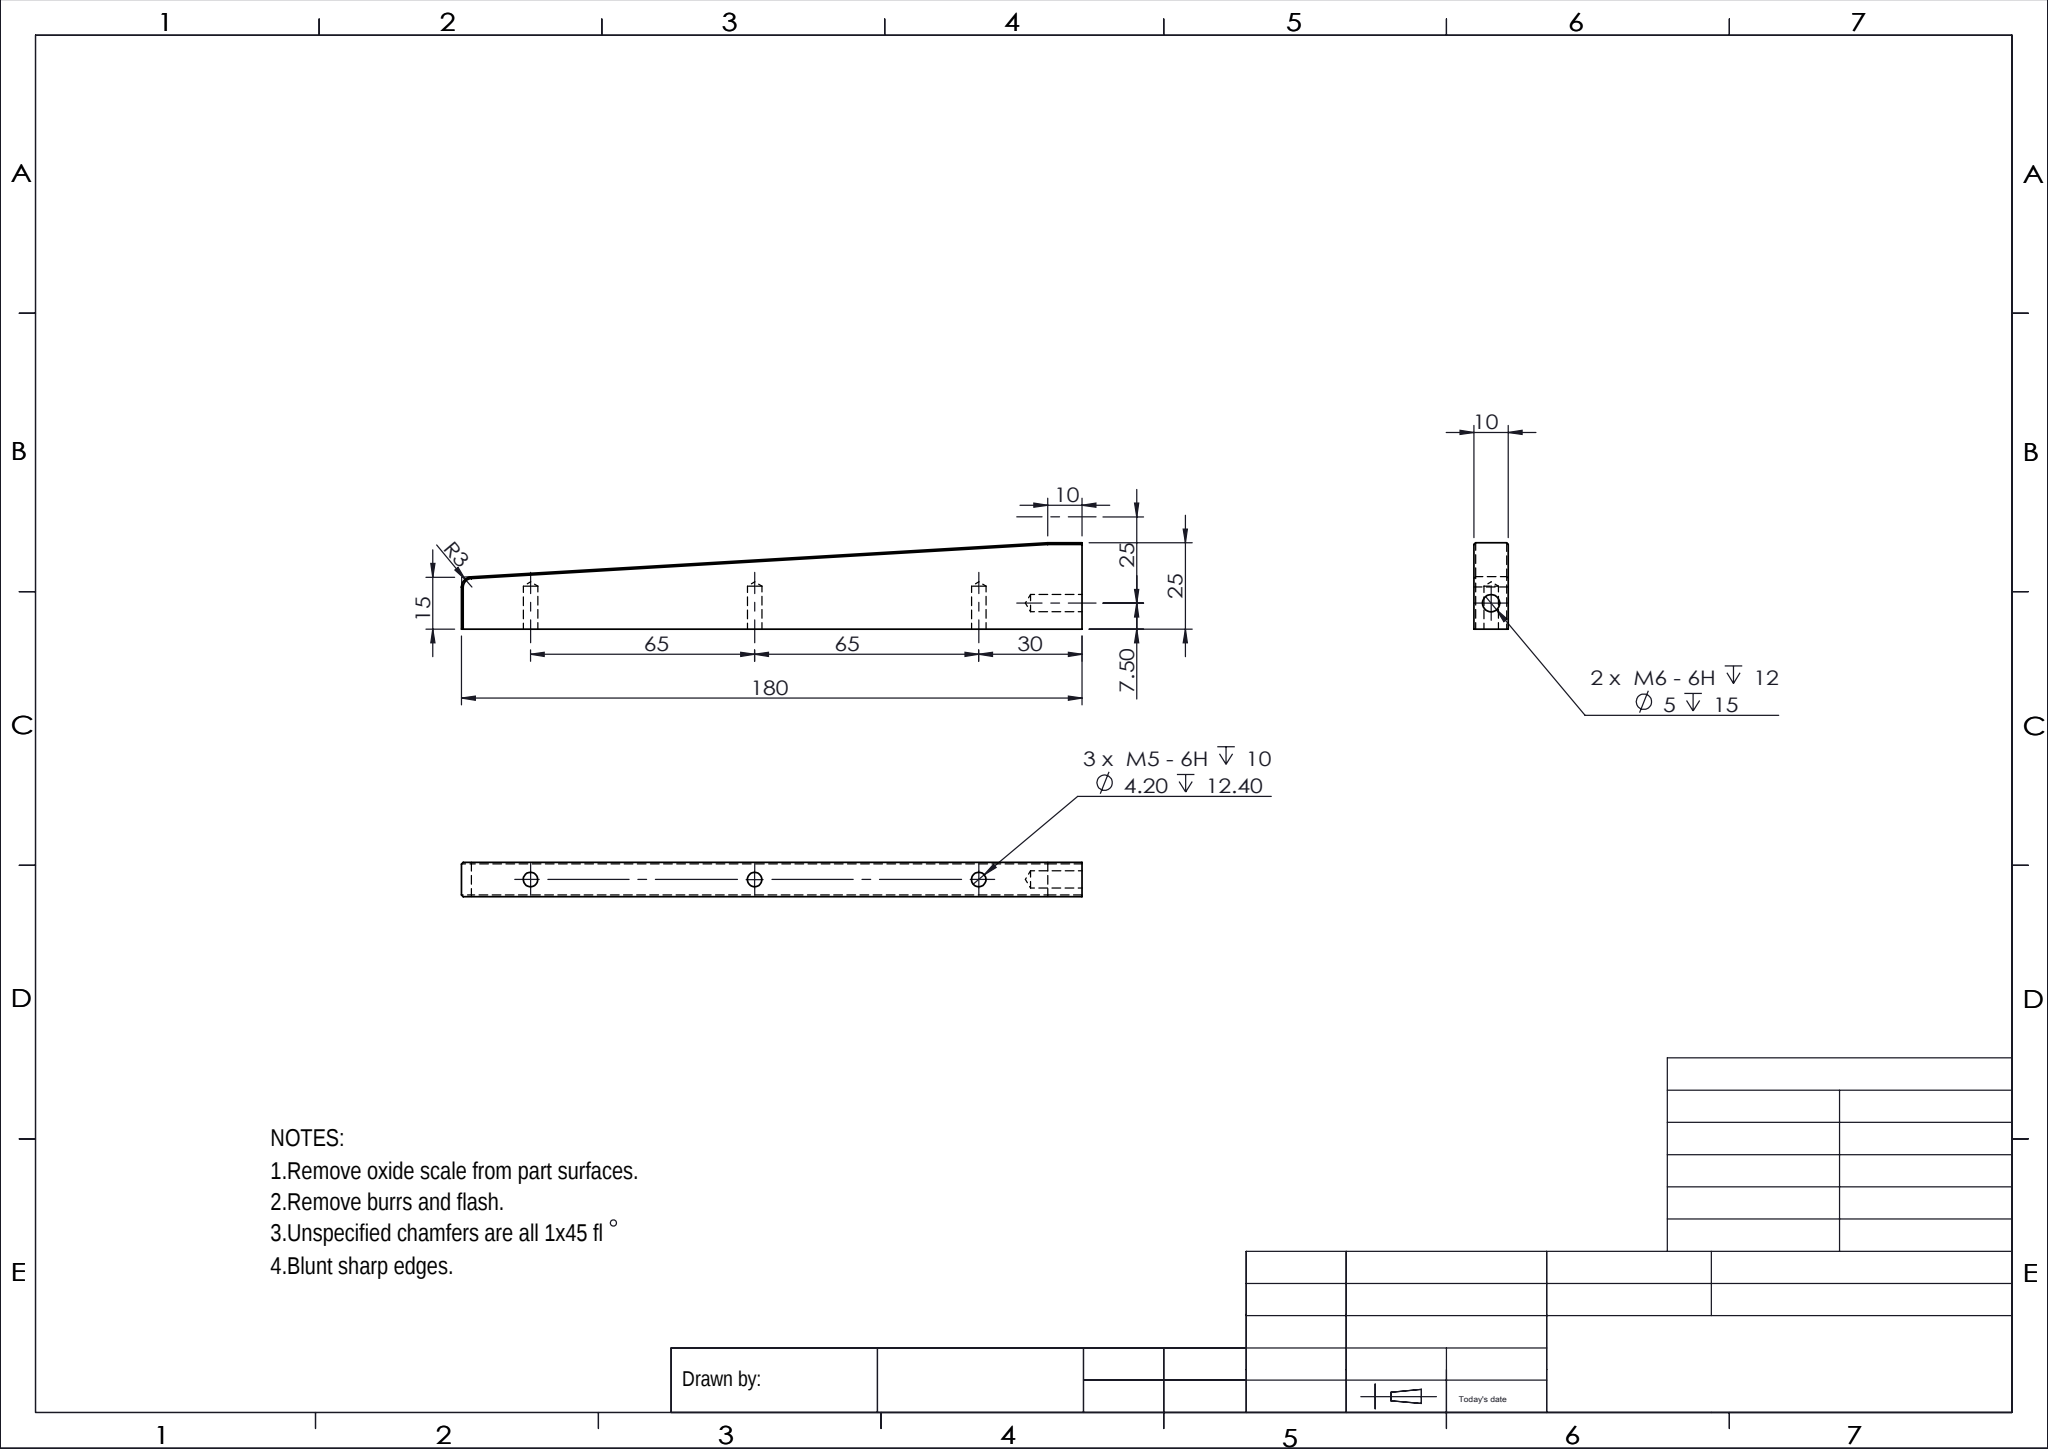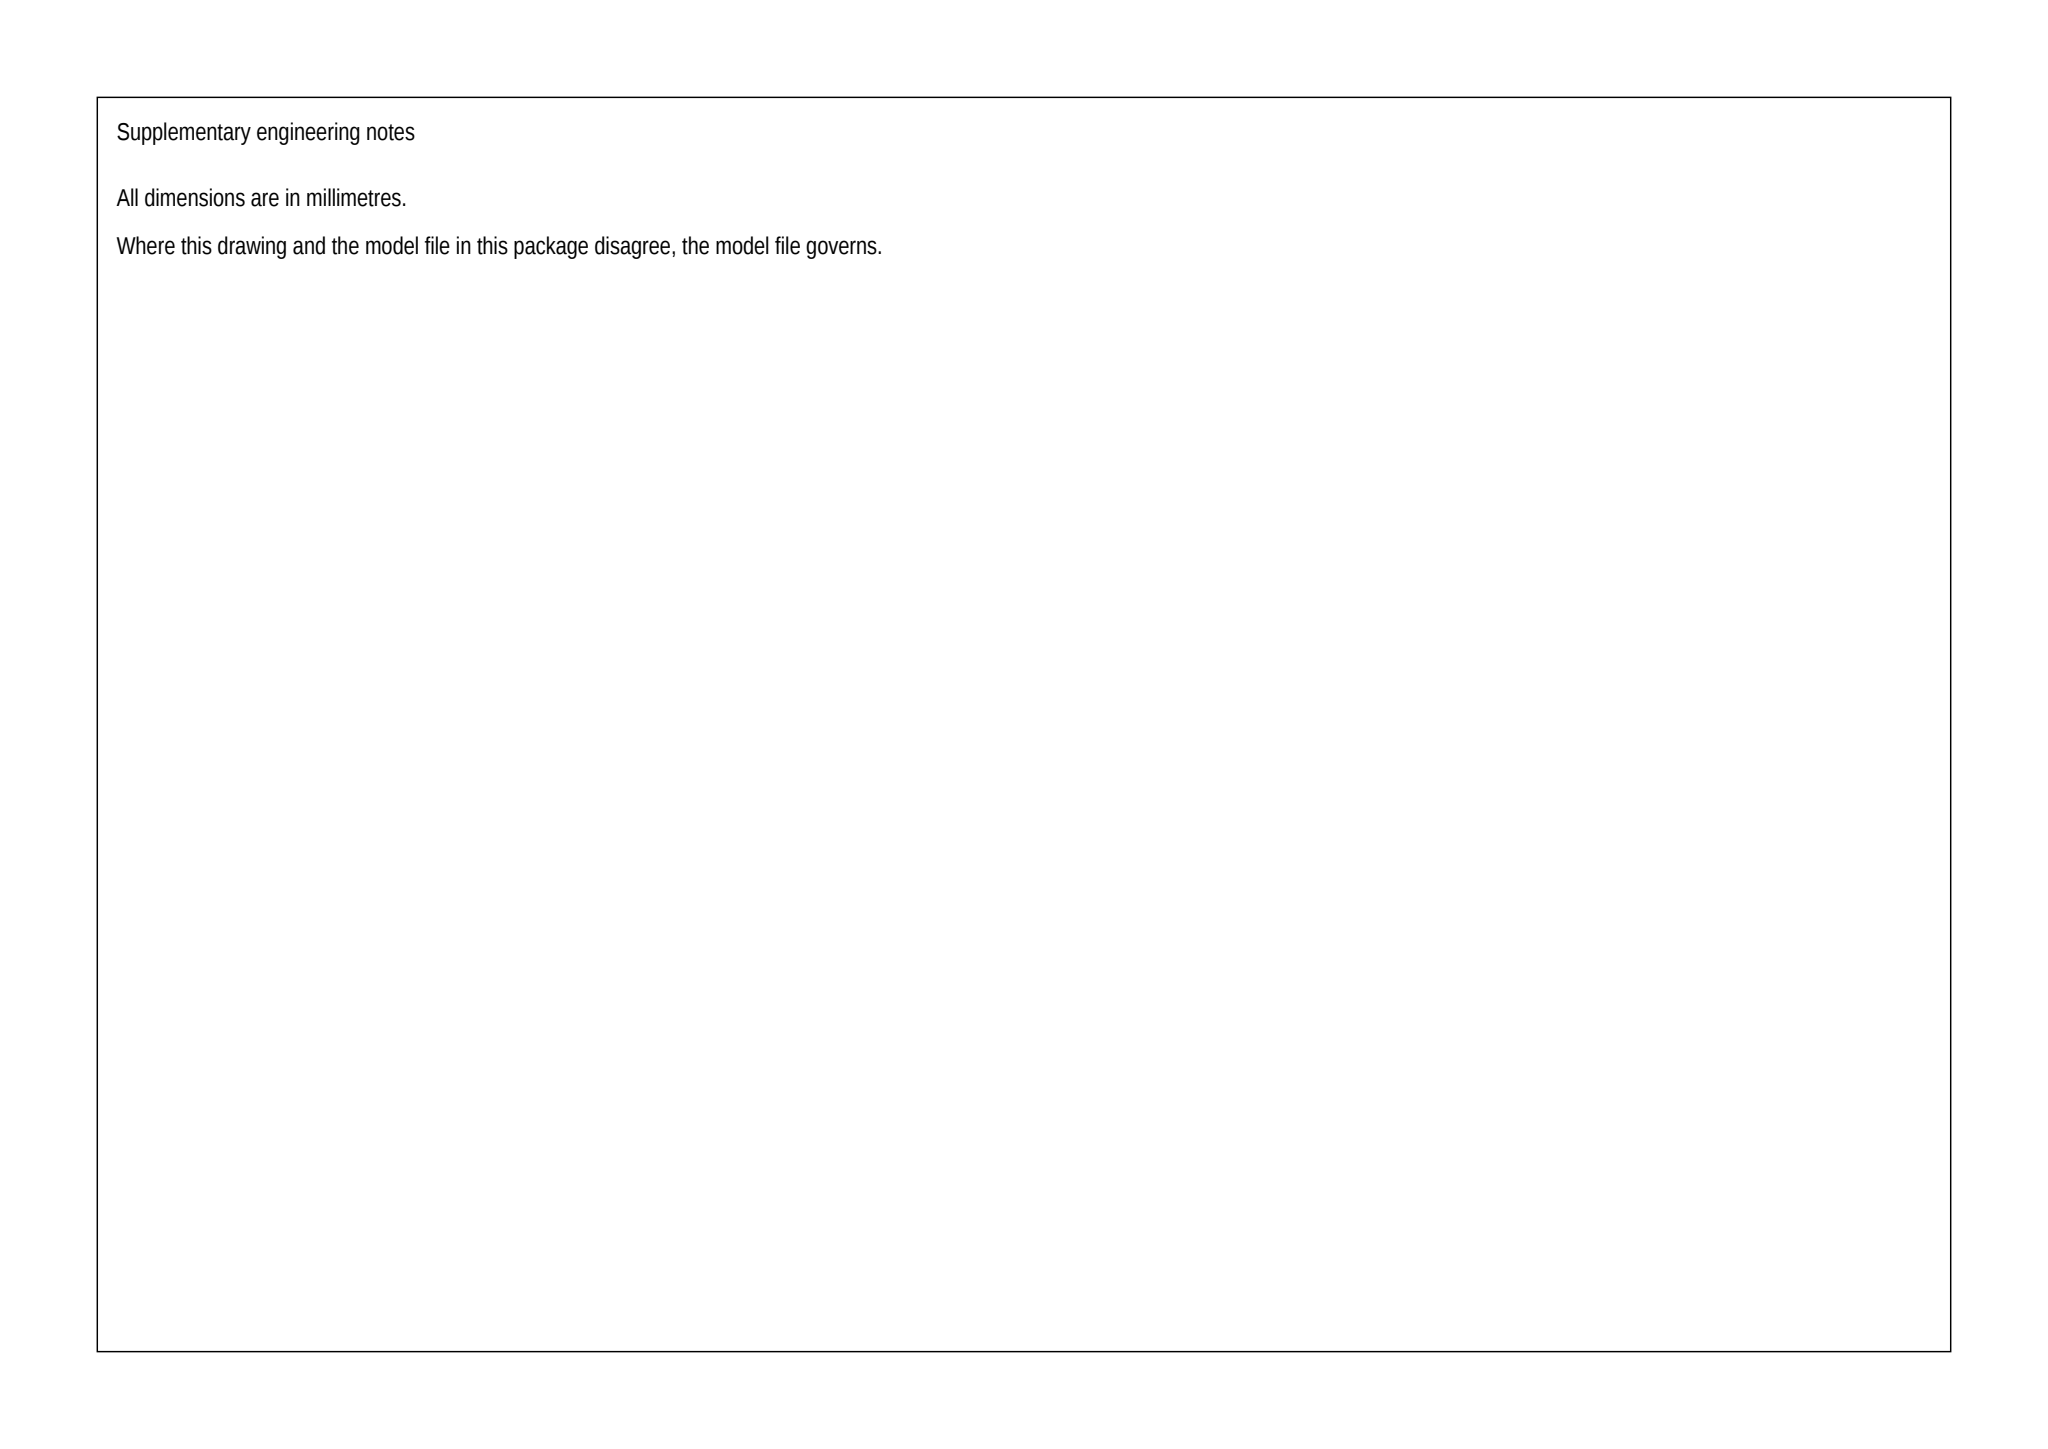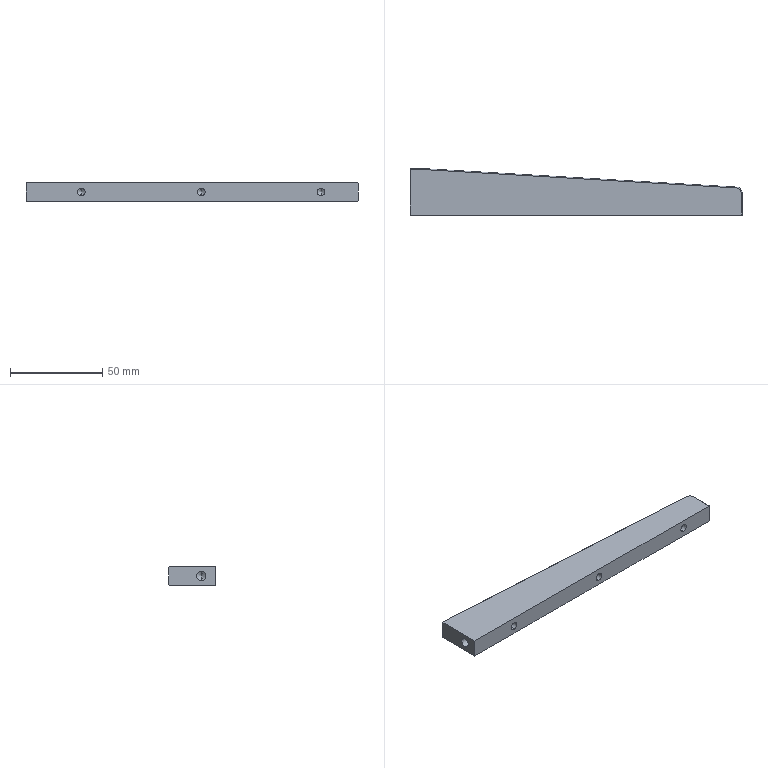Part | SolidWorks | mm | 1 solid | 32 faces | box 180 x 25 x 10 mm | volume 35597 mm3 | plane 13 | cone 10 | cylinder 9 | commonest cylinder face diameters 4.2 x6 5 x2 6 x1
Drawing notes:
UNSPECIFIED CHAMFERS: C0.5 (0.5 X 45°) ALL OVER | from the solid: Inclined planes at 45° with 0.5 x 0.5 section on all edges (e.g. bbox_from [179.5,0,0] size [0.5,12.2,0.5])
NOTE 3 READS: UNSPECIFIED CHAMFERS 0.5 X 45° - NOT 1 X 45° | from the solid: All chamfer faces measure 0.5 leg at 45.0°; no 1.0 chamfers in model
M6 TAPPED HOLE: 1 PL ONLY - QTY IS 1 X, NOT 2 X | from the solid: Only one Ø5 hole on x-axis, from x=0.0 to 15.0 at [y 7.5, z 5.0]
1 X M6-6H DP 12, Ø5 DP 15 IN 25 HIGH END FACE, CL 7.50 FROM BTM | from the solid: Ø5 bore axis x at y=7.5 from bottom face y=0; end face x=0 extent y 0-25
M6 HOLE CTRD IN 10 THK: CL 5.00 FROM EA SIDE FACE | from the solid: Ø5 bore axis at z=5.0 of 10.0 thk (z planes at 0 and 10)
build123d program:
from build123d import *

# Parameters (mm, degrees)
BOSS_EXTRUDE1_DEPTH   = 10
M6_TAPPED_HOLE1_D     = 5
M6_TAPPED_HOLE1_DEPTH = 15
M6_TAPPED_HOLE1_TIP   = 1.502
LPATTERN1_COUNT       = 3
LPATTERN1_PITCH       = 65
FILLET1_R             = 3
CHAMFER1_SIZE         = 0.5


with BuildPart() as part:
    # Sketch1 → Boss-Extrude1 (new body)
    with BuildSketch(Plane.XY):
        Polygon((180, 15), (10, 25), (0, 25), (0, 0), (180, 0), align=None)
    extrude(amount=BOSS_EXTRUDE1_DEPTH)

    # M6 Tapped Hole1
    with Locations(Plane.ZY):
        with Locations((5, 32.5), (5, 7.5)):
            Hole(M6_TAPPED_HOLE1_D / 2, depth=M6_TAPPED_HOLE1_DEPTH)
            with Locations((0, 0, -(M6_TAPPED_HOLE1_DEPTH + M6_TAPPED_HOLE1_TIP / 2))):  # 118° drill point
                Cone(0, M6_TAPPED_HOLE1_D / 2, M6_TAPPED_HOLE1_TIP, mode=Mode.SUBTRACT)

    # Sketch4 → M5 Tapped Hole1 (revolve, cut)
    with BuildSketch(Plane(origin=(30, 0, 5), x_dir=(0, 0, -1), z_dir=(1, 0, 0))):
        Polygon((0, 0), (0, 13.662), (2.1, 12.4), (2.1, 0), align=None)
    m5_tapped_hole1 = revolve(axis=Axis((30, -6.35, 5), (0, 1, 0)), mode=Mode.SUBTRACT)

    # LPattern1: M5 Tapped Hole1 ×3
    with Locations(*[(i * LPATTERN1_PITCH, 0, 0) for i in range(1, LPATTERN1_COUNT)]):
        add(m5_tapped_hole1, mode=Mode.SUBTRACT)

    # Fillet1
    fillet1_edges = [part.edges().sort_by_distance(p)[0] for p in [
        (180, 15, 5),
    ]]
    fillet(fillet1_edges, radius=FILLET1_R)

    # Chamfer1
    chamfer1_edges = [part.edges().sort_by_distance(p)[0] for p in [
        (180, 6.086, 10),
        (5, 25, 10),
        (93.588, 20.083, 0),
        (93.588, 20.083, 10),
        (179.183, 14.229, 0),
        (179.183, 14.229, 10),
        (5, 25, 0),
        (180, 6.086, 0),
    ]]
    chamfer(chamfer1_edges, length=CHAMFER1_SIZE)


solid = part.part
STEP:
#1=CARTESIAN_POINT('',(160.,13.662,5.));
#2=VERTEX_POINT('',#1);
#3=CARTESIAN_POINT('',(160.,12.4,2.9));
#4=VERTEX_POINT('',#3);
#5=CARTESIAN_POINT('',(160.,12.4,2.9));
#6=DIRECTION('',(0.,-0.515,-0.8572));
#7=VECTOR('',#6,1000.);
#8=LINE('',#5,#7);
#9=EDGE_CURVE('',#2,#4,#8,.T.);
#10=ORIENTED_EDGE('',*,*,#9,.F.);
#11=CARTESIAN_POINT('',(160.,12.4,7.1));
#12=VERTEX_POINT('',#11);
#13=CARTESIAN_POINT('',(160.,12.4,7.1));
#14=DIRECTION('',(0.,-0.515,0.8572));
#15=VECTOR('',#14,1000.);
#16=LINE('',#13,#15);
#17=EDGE_CURVE('',#2,#12,#16,.T.);
#18=ORIENTED_EDGE('',*,*,#17,.T.);
#19=CARTESIAN_POINT('',(160.,12.4,5.));
#20=DIRECTION('',(0.,-1.,0.));
#21=DIRECTION('',(0.,0.,-1.));
#22=AXIS2_PLACEMENT_3D('',#19,#20,#21);
#23=CIRCLE('',#22,2.1);
#24=EDGE_CURVE('',#12,#4,#23,.T.);
#25=ORIENTED_EDGE('',*,*,#24,.T.);
#26=EDGE_LOOP('',(#10,#18,#25));
#27=FACE_OUTER_BOUND('',#26,.T.);
#28=CARTESIAN_POINT('',(160.,12.4,5.));
#29=DIRECTION('',(0.,-1.,0.));
#30=DIRECTION('',(0.,0.,-1.));
#31=AXIS2_PLACEMENT_3D('',#28,#29,#30);
#32=CONICAL_SURFACE('',#31,2.1,1.03);
#33=ADVANCED_FACE('',(#27),#32,.F.);
#34=ORIENTED_EDGE('',*,*,#24,.F.);
#35=CARTESIAN_POINT('',(160.,-0.,7.1));
#36=VERTEX_POINT('',#35);
#37=CARTESIAN_POINT('',(160.,0.,7.1));
#38=DIRECTION('',(0.,-1.,0.));
#39=VECTOR('',#38,1000.);
#40=LINE('',#37,#39);
#41=EDGE_CURVE('',#12,#36,#40,.T.);
#42=ORIENTED_EDGE('',*,*,#41,.T.);
#43=CARTESIAN_POINT('',(160.,-0.,2.9));
#44=VERTEX_POINT('',#43);
#45=CARTESIAN_POINT('',(160.,-0.,5.));
#46=DIRECTION('',(0.,-1.,0.));
#47=DIRECTION('',(0.,0.,-1.));
#48=AXIS2_PLACEMENT_3D('',#45,#46,#47);
#49=CIRCLE('',#48,2.1);
#50=EDGE_CURVE('',#36,#44,#49,.T.);
#51=ORIENTED_EDGE('',*,*,#50,.T.);
#52=CARTESIAN_POINT('',(160.,0.,2.9));
#53=DIRECTION('',(0.,-1.,0.));
#54=VECTOR('',#53,1000.);
#55=LINE('',#52,#54);
#56=EDGE_CURVE('',#4,#44,#55,.T.);
#57=ORIENTED_EDGE('',*,*,#56,.F.);
#58=EDGE_LOOP('',(#34,#42,#51,#57));
#59=FACE_OUTER_BOUND('',#58,.T.);
#60=CARTESIAN_POINT('',(160.,0.,5.));
#61=DIRECTION('',(0.,-1.,0.));
#62=DIRECTION('',(0.,0.,-1.));
#63=AXIS2_PLACEMENT_3D('',#60,#61,#62);
#64=CYLINDRICAL_SURFACE('',#63,2.1);
#65=ADVANCED_FACE('',(#59),#64,.F.);
#66=CARTESIAN_POINT('',(95.,12.4,7.1));
#67=VERTEX_POINT('',#66);
#68=CARTESIAN_POINT('',(95.,12.4,2.9));
#69=VERTEX_POINT('',#68);
#70=CARTESIAN_POINT('',(95.,12.4,5.));
#71=DIRECTION('',(0.,-1.,0.));
#72=DIRECTION('',(0.,0.,-1.));
#73=AXIS2_PLACEMENT_3D('',#70,#71,#72);
#74=CIRCLE('',#73,2.1);
#75=EDGE_CURVE('',#67,#69,#74,.T.);
#76=ORIENTED_EDGE('',*,*,#75,.F.);
#77=CARTESIAN_POINT('',(95.,-0.,7.1));
#78=VERTEX_POINT('',#77);
#79=CARTESIAN_POINT('',(95.,0.,7.1));
#80=DIRECTION('',(0.,-1.,0.));
#81=VECTOR('',#80,1000.);
#82=LINE('',#79,#81);
#83=EDGE_CURVE('',#67,#78,#82,.T.);
#84=ORIENTED_EDGE('',*,*,#83,.T.);
#85=CARTESIAN_POINT('',(95.,-0.,2.9));
#86=VERTEX_POINT('',#85);
#87=CARTESIAN_POINT('',(95.,-0.,5.));
#88=DIRECTION('',(0.,-1.,0.));
#89=DIRECTION('',(0.,0.,-1.));
#90=AXIS2_PLACEMENT_3D('',#87,#88,#89);
#91=CIRCLE('',#90,2.1);
#92=EDGE_CURVE('',#78,#86,#91,.T.);
#93=ORIENTED_EDGE('',*,*,#92,.T.);
#94=CARTESIAN_POINT('',(95.,0.,2.9));
#95=DIRECTION('',(0.,-1.,0.));
#96=VECTOR('',#95,1000.);
#97=LINE('',#94,#96);
#98=EDGE_CURVE('',#69,#86,#97,.T.);
#99=ORIENTED_EDGE('',*,*,#98,.F.);
#100=EDGE_LOOP('',(#76,#84,#93,#99));
#101=FACE_OUTER_BOUND('',#100,.T.);
#102=CARTESIAN_POINT('',(95.,0.,5.));
#103=DIRECTION('',(0.,-1.,0.));
#104=DIRECTION('',(0.,0.,-1.));
#105=AXIS2_PLACEMENT_3D('',#102,#103,#104);
#106=CYLINDRICAL_SURFACE('',#105,2.1);
#107=ADVANCED_FACE('',(#101),#106,.F.);
#108=CARTESIAN_POINT('',(95.,13.662,5.));
#109=VERTEX_POINT('',#108);
#110=CARTESIAN_POINT('',(95.,12.4,2.9));
#111=DIRECTION('',(0.,-0.515,-0.8572));
#112=VECTOR('',#111,1000.);
#113=LINE('',#110,#112);
#114=EDGE_CURVE('',#109,#69,#113,.T.);
#115=ORIENTED_EDGE('',*,*,#114,.F.);
#116=CARTESIAN_POINT('',(95.,12.4,7.1));
#117=DIRECTION('',(0.,-0.515,0.8572));
#118=VECTOR('',#117,1000.);
#119=LINE('',#116,#118);
#120=EDGE_CURVE('',#109,#67,#119,.T.);
#121=ORIENTED_EDGE('',*,*,#120,.T.);
#122=ORIENTED_EDGE('',*,*,#75,.T.);
#123=EDGE_LOOP('',(#115,#121,#122));
#124=FACE_OUTER_BOUND('',#123,.T.);
#125=CARTESIAN_POINT('',(95.,12.4,5.));
#126=DIRECTION('',(0.,-1.,0.));
#127=DIRECTION('',(0.,0.,-1.));
#128=AXIS2_PLACEMENT_3D('',#125,#126,#127);
#129=CONICAL_SURFACE('',#128,2.1,1.03);
#130=ADVANCED_FACE('',(#124),#129,.F.);
#131=CARTESIAN_POINT('',(30.,12.4,7.1));
#132=VERTEX_POINT('',#131);
#133=CARTESIAN_POINT('',(30.,12.4,2.9));
#134=VERTEX_POINT('',#133);
#135=CARTESIAN_POINT('',(30.,12.4,5.));
#136=DIRECTION('',(0.,-1.,0.));
#137=DIRECTION('',(0.,0.,-1.));
#138=AXIS2_PLACEMENT_3D('',#135,#136,#137);
#139=CIRCLE('',#138,2.1);
#140=EDGE_CURVE('',#132,#134,#139,.T.);
#141=ORIENTED_EDGE('',*,*,#140,.F.);
#142=CARTESIAN_POINT('',(30.,-0.,7.1));
#143=VERTEX_POINT('',#142);
#144=CARTESIAN_POINT('',(30.,0.,7.1));
#145=DIRECTION('',(0.,-1.,0.));
#146=VECTOR('',#145,1000.);
#147=LINE('',#144,#146);
#148=EDGE_CURVE('',#132,#143,#147,.T.);
#149=ORIENTED_EDGE('',*,*,#148,.T.);
#150=CARTESIAN_POINT('',(30.,-0.,2.9));
#151=VERTEX_POINT('',#150);
#152=CARTESIAN_POINT('',(30.,-0.,5.));
#153=DIRECTION('',(0.,-1.,0.));
#154=DIRECTION('',(0.,0.,-1.));
#155=AXIS2_PLACEMENT_3D('',#152,#153,#154);
#156=CIRCLE('',#155,2.1);
#157=EDGE_CURVE('',#143,#151,#156,.T.);
#158=ORIENTED_EDGE('',*,*,#157,.T.);
#159=CARTESIAN_POINT('',(30.,0.,2.9));
#160=DIRECTION('',(0.,-1.,0.));
#161=VECTOR('',#160,1000.);
#162=LINE('',#159,#161);
#163=EDGE_CURVE('',#134,#151,#162,.T.);
#164=ORIENTED_EDGE('',*,*,#163,.F.);
#165=EDGE_LOOP('',(#141,#149,#158,#164));
#166=FACE_OUTER_BOUND('',#165,.T.);
#167=CARTESIAN_POINT('',(30.,0.,5.));
#168=DIRECTION('',(0.,-1.,0.));
#169=DIRECTION('',(0.,0.,-1.));
#170=AXIS2_PLACEMENT_3D('',#167,#168,#169);
#171=CYLINDRICAL_SURFACE('',#170,2.1);
#172=ADVANCED_FACE('',(#166),#171,.F.);
#173=CARTESIAN_POINT('',(30.,13.662,5.));
#174=VERTEX_POINT('',#173);
#175=CARTESIAN_POINT('',(30.,12.4,2.9));
#176=DIRECTION('',(0.,-0.515,-0.8572));
#177=VECTOR('',#176,1000.);
#178=LINE('',#175,#177);
#179=EDGE_CURVE('',#174,#134,#178,.T.);
#180=ORIENTED_EDGE('',*,*,#179,.F.);
#181=CARTESIAN_POINT('',(30.,12.4,7.1));
#182=DIRECTION('',(0.,-0.515,0.8572));
#183=VECTOR('',#182,1000.);
#184=LINE('',#181,#183);
#185=EDGE_CURVE('',#174,#132,#184,.T.);
#186=ORIENTED_EDGE('',*,*,#185,.T.);
#187=ORIENTED_EDGE('',*,*,#140,.T.);
#188=EDGE_LOOP('',(#180,#186,#187));
#189=FACE_OUTER_BOUND('',#188,.T.);
#190=CARTESIAN_POINT('',(30.,12.4,5.));
#191=DIRECTION('',(0.,-1.,0.));
#192=DIRECTION('',(0.,0.,-1.));
#193=AXIS2_PLACEMENT_3D('',#190,#191,#192);
#194=CONICAL_SURFACE('',#193,2.1,1.03);
#195=ADVANCED_FACE('',(#189),#194,.F.);
#196=CARTESIAN_POINT('',(15.,7.5,2.5));
#197=VERTEX_POINT('',#196);
#198=CARTESIAN_POINT('',(15.,7.5,7.5));
#199=VERTEX_POINT('',#198);
#200=CARTESIAN_POINT('',(15.,7.5,5.));
#201=DIRECTION('',(-1.,0.,0.));
#202=DIRECTION('',(0.,0.,1.));
#203=AXIS2_PLACEMENT_3D('',#200,#201,#202);
#204=CIRCLE('',#203,2.5);
#205=EDGE_CURVE('',#197,#199,#204,.T.);
#206=ORIENTED_EDGE('',*,*,#205,.F.);
#207=CARTESIAN_POINT('',(-0.,7.5,2.5));
#208=VERTEX_POINT('',#207);
#209=CARTESIAN_POINT('',(0.,7.5,2.5));
#210=DIRECTION('',(-1.,0.,0.));
#211=VECTOR('',#210,1000.);
#212=LINE('',#209,#211);
#213=EDGE_CURVE('',#197,#208,#212,.T.);
#214=ORIENTED_EDGE('',*,*,#213,.T.);
#215=CARTESIAN_POINT('',(-0.,7.5,7.5));
#216=VERTEX_POINT('',#215);
#217=CARTESIAN_POINT('',(-0.,7.5,5.));
#218=DIRECTION('',(-1.,0.,0.));
#219=DIRECTION('',(0.,0.,1.));
#220=AXIS2_PLACEMENT_3D('',#217,#218,#219);
#221=CIRCLE('',#220,2.5);
#222=EDGE_CURVE('',#208,#216,#221,.T.);
#223=ORIENTED_EDGE('',*,*,#222,.T.);
#224=CARTESIAN_POINT('',(0.,7.5,7.5));
#225=DIRECTION('',(-1.,0.,0.));
#226=VECTOR('',#225,1000.);
#227=LINE('',#224,#226);
#228=EDGE_CURVE('',#199,#216,#227,.T.);
#229=ORIENTED_EDGE('',*,*,#228,.F.);
#230=EDGE_LOOP('',(#206,#214,#223,#229));
#231=FACE_OUTER_BOUND('',#230,.T.);
#232=CARTESIAN_POINT('',(0.,7.5,5.));
#233=DIRECTION('',(-1.,0.,0.));
#234=DIRECTION('',(0.,0.,1.));
#235=AXIS2_PLACEMENT_3D('',#232,#233,#234);
#236=CYLINDRICAL_SURFACE('',#235,2.5);
#237=ADVANCED_FACE('',(#231),#236,.F.);
#238=CARTESIAN_POINT('',(16.502,7.5,5.));
#239=VERTEX_POINT('',#238);
#240=CARTESIAN_POINT('',(15.,7.5,7.5));
#241=DIRECTION('',(-0.515,0.,0.8572));
#242=VECTOR('',#241,1000.);
#243=LINE('',#240,#242);
#244=EDGE_CURVE('',#239,#199,#243,.T.);
#245=ORIENTED_EDGE('',*,*,#244,.F.);
#246=CARTESIAN_POINT('',(15.,7.5,2.5));
#247=DIRECTION('',(-0.515,0.,-0.8572));
#248=VECTOR('',#247,1000.);
#249=LINE('',#246,#248);
#250=EDGE_CURVE('',#239,#197,#249,.T.);
#251=ORIENTED_EDGE('',*,*,#250,.T.);
#252=ORIENTED_EDGE('',*,*,#205,.T.);
#253=EDGE_LOOP('',(#245,#251,#252));
#254=FACE_OUTER_BOUND('',#253,.T.);
#255=CARTESIAN_POINT('',(15.,7.5,5.));
#256=DIRECTION('',(-1.,0.,0.));
#257=DIRECTION('',(0.,0.,1.));
#258=AXIS2_PLACEMENT_3D('',#255,#256,#257);
#259=CONICAL_SURFACE('',#258,2.5,1.03);
#260=ADVANCED_FACE('',(#254),#259,.F.);
#261=CARTESIAN_POINT('',(-0.,7.5,5.));
#262=DIRECTION('',(-1.,0.,0.));
#263=DIRECTION('',(0.,0.,1.));
#264=AXIS2_PLACEMENT_3D('',#261,#262,#263);
#265=CIRCLE('',#264,2.5);
#266=EDGE_CURVE('',#216,#208,#265,.T.);
#267=ORIENTED_EDGE('',*,*,#266,.F.);
#268=ORIENTED_EDGE('',*,*,#222,.F.);
#269=EDGE_LOOP('',(#267,#268));
#270=FACE_BOUND('',#269,.T.);
#271=CARTESIAN_POINT('',(0.,24.5,10.));
#272=VERTEX_POINT('',#271);
#273=CARTESIAN_POINT('',(0.,0.,10.));
#274=VERTEX_POINT('',#273);
#275=CARTESIAN_POINT('',(0.,0.,10.));
#276=DIRECTION('',(0.,-1.,0.));
#277=VECTOR('',#276,1000.);
#278=LINE('',#275,#277);
#279=EDGE_CURVE('',#272,#274,#278,.T.);
#280=ORIENTED_EDGE('',*,*,#279,.F.);
#281=CARTESIAN_POINT('',(0.,25.,9.5));
#282=VERTEX_POINT('',#281);
#283=CARTESIAN_POINT('',(0.,24.5,10.));
#284=DIRECTION('',(0.,0.7071,-0.7071));
#285=VECTOR('',#284,1000.);
#286=LINE('',#283,#285);
#287=EDGE_CURVE('',#272,#282,#286,.T.);
#288=ORIENTED_EDGE('',*,*,#287,.T.);
#289=CARTESIAN_POINT('',(0.,25.,0.5));
#290=VERTEX_POINT('',#289);
#291=CARTESIAN_POINT('',(0.,25.,10.));
#292=DIRECTION('',(0.,0.,-1.));
#293=VECTOR('',#292,1000.);
#294=LINE('',#291,#293);
#295=EDGE_CURVE('',#282,#290,#294,.T.);
#296=ORIENTED_EDGE('',*,*,#295,.T.);
#297=CARTESIAN_POINT('',(0.,24.5,0.));
#298=VERTEX_POINT('',#297);
#299=CARTESIAN_POINT('',(0.,25.,0.5));
#300=DIRECTION('',(0.,-0.7071,-0.7071));
#301=VECTOR('',#300,1000.);
#302=LINE('',#299,#301);
#303=EDGE_CURVE('',#290,#298,#302,.T.);
#304=ORIENTED_EDGE('',*,*,#303,.T.);
#305=CARTESIAN_POINT('',(0.,0.,0.));
#306=VERTEX_POINT('',#305);
#307=CARTESIAN_POINT('',(0.,0.,0.));
#308=DIRECTION('',(0.,-1.,0.));
#309=VECTOR('',#308,1000.);
#310=LINE('',#307,#309);
#311=EDGE_CURVE('',#298,#306,#310,.T.);
#312=ORIENTED_EDGE('',*,*,#311,.T.);
#313=CARTESIAN_POINT('',(0.,0.,10.));
#314=DIRECTION('',(0.,0.,-1.));
#315=VECTOR('',#314,1000.);
#316=LINE('',#313,#315);
#317=EDGE_CURVE('',#274,#306,#316,.T.);
#318=ORIENTED_EDGE('',*,*,#317,.F.);
#319=EDGE_LOOP('',(#280,#288,#296,#304,#312,#318));
#320=FACE_OUTER_BOUND('',#319,.T.);
#321=CARTESIAN_POINT('',(0.,0.,10.));
#322=DIRECTION('',(1.,0.,0.));
#323=DIRECTION('',(0.,0.,-1.));
#324=AXIS2_PLACEMENT_3D('',#321,#322,#323);
#325=PLANE('',#324);
#326=ADVANCED_FACE('',(#270,#320),#325,.F.);
#327=CARTESIAN_POINT('',(95.,-0.,5.));
#328=DIRECTION('',(0.,-1.,0.));
#329=DIRECTION('',(0.,0.,-1.));
#330=AXIS2_PLACEMENT_3D('',#327,#328,#329);
#331=CIRCLE('',#330,2.1);
#332=EDGE_CURVE('',#86,#78,#331,.T.);
#333=ORIENTED_EDGE('',*,*,#332,.F.);
#334=ORIENTED_EDGE('',*,*,#92,.F.);
#335=EDGE_LOOP('',(#333,#334));
#336=FACE_BOUND('',#335,.T.);
#337=CARTESIAN_POINT('',(30.,-0.,5.));
#338=DIRECTION('',(0.,-1.,0.));
#339=DIRECTION('',(0.,0.,-1.));
#340=AXIS2_PLACEMENT_3D('',#337,#338,#339);
#341=CIRCLE('',#340,2.1);
#342=EDGE_CURVE('',#151,#143,#341,.T.);
#343=ORIENTED_EDGE('',*,*,#342,.F.);
#344=ORIENTED_EDGE('',*,*,#157,.F.);
#345=EDGE_LOOP('',(#343,#344));
#346=FACE_BOUND('',#345,.T.);
#347=CARTESIAN_POINT('',(180.,0.,9.5));
#348=VERTEX_POINT('',#347);
#349=CARTESIAN_POINT('',(180.,0.,0.5));
#350=VERTEX_POINT('',#349);
#351=CARTESIAN_POINT('',(180.,0.,10.));
#352=DIRECTION('',(0.,0.,-1.));
#353=VECTOR('',#352,1000.);
#354=LINE('',#351,#353);
#355=EDGE_CURVE('',#348,#350,#354,.T.);
#356=ORIENTED_EDGE('',*,*,#355,.F.);
#357=CARTESIAN_POINT('',(179.5,0.,10.));
#358=VERTEX_POINT('',#357);
#359=CARTESIAN_POINT('',(179.5,0.,10.));
#360=DIRECTION('',(-0.7071,0.,0.7071));
#361=VECTOR('',#360,1000.);
#362=LINE('',#359,#361);
#363=EDGE_CURVE('',#348,#358,#362,.T.);
#364=ORIENTED_EDGE('',*,*,#363,.T.);
#365=CARTESIAN_POINT('',(0.,0.,10.));
#366=DIRECTION('',(1.,0.,0.));
#367=VECTOR('',#366,1000.);
#368=LINE('',#365,#367);
#369=EDGE_CURVE('',#274,#358,#368,.T.);
#370=ORIENTED_EDGE('',*,*,#369,.F.);
#371=ORIENTED_EDGE('',*,*,#317,.T.);
#372=CARTESIAN_POINT('',(179.5,0.,-0.));
#373=VERTEX_POINT('',#372);
#374=CARTESIAN_POINT('',(0.,0.,0.));
#375=DIRECTION('',(1.,0.,0.));
#376=VECTOR('',#375,1000.);
#377=LINE('',#374,#376);
#378=EDGE_CURVE('',#306,#373,#377,.T.);
#379=ORIENTED_EDGE('',*,*,#378,.T.);
#380=CARTESIAN_POINT('',(180.,0.,0.5));
#381=DIRECTION('',(0.7071,0.,0.7071));
#382=VECTOR('',#381,1000.);
#383=LINE('',#380,#382);
#384=EDGE_CURVE('',#373,#350,#383,.T.);
#385=ORIENTED_EDGE('',*,*,#384,.T.);
#386=EDGE_LOOP('',(#356,#364,#370,#371,#379,#385));
#387=FACE_OUTER_BOUND('',#386,.T.);
#388=CARTESIAN_POINT('',(160.,-0.,5.));
#389=DIRECTION('',(0.,-1.,0.));
#390=DIRECTION('',(0.,0.,-1.));
#391=AXIS2_PLACEMENT_3D('',#388,#389,#390);
#392=CIRCLE('',#391,2.1);
#393=EDGE_CURVE('',#44,#36,#392,.T.);
#394=ORIENTED_EDGE('',*,*,#393,.F.);
#395=ORIENTED_EDGE('',*,*,#50,.F.);
#396=EDGE_LOOP('',(#394,#395));
#397=FACE_BOUND('',#396,.T.);
#398=CARTESIAN_POINT('',(0.,0.,10.));
#399=DIRECTION('',(0.,1.,0.));
#400=DIRECTION('',(0.,0.,1.));
#401=AXIS2_PLACEMENT_3D('',#398,#399,#400);
#402=PLANE('',#401);
#403=ADVANCED_FACE('',(#336,#346,#387,#397),#402,.F.);
#404=CARTESIAN_POINT('',(180.,12.171,0.5));
#405=VERTEX_POINT('',#404);
#406=CARTESIAN_POINT('',(180.,12.171,9.5));
#407=VERTEX_POINT('',#406);
#408=CARTESIAN_POINT('',(180.,12.171,10.));
#409=DIRECTION('',(0.,0.,1.));
#410=VECTOR('',#409,1000.);
#411=LINE('',#408,#410);
#412=EDGE_CURVE('',#405,#407,#411,.T.);
#413=ORIENTED_EDGE('',*,*,#412,.T.);
#414=CARTESIAN_POINT('',(180.,0.,9.5));
#415=DIRECTION('',(0.,-1.,0.));
#416=VECTOR('',#415,1000.);
#417=LINE('',#414,#416);
#418=EDGE_CURVE('',#407,#348,#417,.T.);
#419=ORIENTED_EDGE('',*,*,#418,.T.);
#420=ORIENTED_EDGE('',*,*,#355,.T.);
#421=CARTESIAN_POINT('',(180.,12.171,0.5));
#422=DIRECTION('',(0.,1.,0.));
#423=VECTOR('',#422,1000.);
#424=LINE('',#421,#423);
#425=EDGE_CURVE('',#350,#405,#424,.T.);
#426=ORIENTED_EDGE('',*,*,#425,.T.);
#427=EDGE_LOOP('',(#413,#419,#420,#426));
#428=FACE_OUTER_BOUND('',#427,.T.);
#429=CARTESIAN_POINT('',(180.,0.,10.));
#430=DIRECTION('',(-1.,0.,0.));
#431=DIRECTION('',(0.,0.,1.));
#432=AXIS2_PLACEMENT_3D('',#429,#430,#431);
#433=PLANE('',#432);
#434=ADVANCED_FACE('',(#428),#433,.F.);
#435=CARTESIAN_POINT('',(10.,25.,9.5));
#436=VERTEX_POINT('',#435);
#437=CARTESIAN_POINT('',(10.,25.,0.5));
#438=VERTEX_POINT('',#437);
#439=CARTESIAN_POINT('',(10.,25.,10.));
#440=DIRECTION('',(0.,0.,-1.));
#441=VECTOR('',#440,1000.);
#442=LINE('',#439,#441);
#443=EDGE_CURVE('',#436,#438,#442,.T.);
#444=ORIENTED_EDGE('',*,*,#443,.F.);
#445=CARTESIAN_POINT('',(177.176,15.166,9.5));
#446=VERTEX_POINT('',#445);
#447=CARTESIAN_POINT('',(180.,15.,9.5));
#448=DIRECTION('',(0.9983,-0.05872,0.));
#449=VECTOR('',#448,1000.);
#450=LINE('',#447,#449);
#451=EDGE_CURVE('',#436,#446,#450,.T.);
#452=ORIENTED_EDGE('',*,*,#451,.T.);
#453=CARTESIAN_POINT('',(177.176,15.166,0.5));
#454=VERTEX_POINT('',#453);
#455=CARTESIAN_POINT('',(177.176,15.166,10.));
#456=DIRECTION('',(0.,0.,-1.));
#457=VECTOR('',#456,1000.);
#458=LINE('',#455,#457);
#459=EDGE_CURVE('',#446,#454,#458,.T.);
#460=ORIENTED_EDGE('',*,*,#459,.T.);
#461=CARTESIAN_POINT('',(10.,25.,0.5));
#462=DIRECTION('',(-0.9983,0.05872,0.));
#463=VECTOR('',#462,1000.);
#464=LINE('',#461,#463);
#465=EDGE_CURVE('',#454,#438,#464,.T.);
#466=ORIENTED_EDGE('',*,*,#465,.T.);
#467=EDGE_LOOP('',(#444,#452,#460,#466));
#468=FACE_OUTER_BOUND('',#467,.T.);
#469=CARTESIAN_POINT('',(180.,15.,10.));
#470=DIRECTION('',(-0.05872,-0.9983,0.));
#471=DIRECTION('',(0.9983,-0.05872,0.));
#472=AXIS2_PLACEMENT_3D('',#469,#470,#471);
#473=PLANE('',#472);
#474=ADVANCED_FACE('',(#468),#473,.F.);
#475=ORIENTED_EDGE('',*,*,#295,.F.);
#476=CARTESIAN_POINT('',(0.,25.,9.5));
#477=DIRECTION('',(1.,0.,0.));
#478=VECTOR('',#477,1000.);
#479=LINE('',#476,#478);
#480=EDGE_CURVE('',#282,#436,#479,.T.);
#481=ORIENTED_EDGE('',*,*,#480,.T.);
#482=ORIENTED_EDGE('',*,*,#443,.T.);
#483=CARTESIAN_POINT('',(0.,25.,0.5));
#484=DIRECTION('',(-1.,0.,0.));
#485=VECTOR('',#484,1000.);
#486=LINE('',#483,#485);
#487=EDGE_CURVE('',#438,#290,#486,.T.);
#488=ORIENTED_EDGE('',*,*,#487,.T.);
#489=EDGE_LOOP('',(#475,#481,#482,#488));
#490=FACE_OUTER_BOUND('',#489,.T.);
#491=CARTESIAN_POINT('',(0.,25.,10.));
#492=DIRECTION('',(0.,-1.,0.));
#493=DIRECTION('',(0.,0.,-1.));
#494=AXIS2_PLACEMENT_3D('',#491,#492,#493);
#495=PLANE('',#494);
#496=ADVANCED_FACE('',(#490),#495,.F.);
#497=CARTESIAN_POINT('',(177.147,14.667,10.));
#498=VERTEX_POINT('',#497);
#499=CARTESIAN_POINT('',(9.985,24.5,10.));
#500=VERTEX_POINT('',#499);
#501=CARTESIAN_POINT('',(1.471,25.001,10.));
#502=DIRECTION('',(-0.9983,0.05872,0.));
#503=VECTOR('',#502,1000.);
#504=LINE('',#501,#503);
#505=EDGE_CURVE('',#498,#500,#504,.T.);
#506=ORIENTED_EDGE('',*,*,#505,.T.);
#507=CARTESIAN_POINT('',(0.,24.5,10.));
#508=DIRECTION('',(-1.,0.,0.));
#509=VECTOR('',#508,1000.);
#510=LINE('',#507,#509);
#511=EDGE_CURVE('',#500,#272,#510,.T.);
#512=ORIENTED_EDGE('',*,*,#511,.T.);
#513=ORIENTED_EDGE('',*,*,#279,.T.);
#514=ORIENTED_EDGE('',*,*,#369,.T.);
#515=CARTESIAN_POINT('',(179.5,12.171,10.));
#516=VERTEX_POINT('',#515);
#517=CARTESIAN_POINT('',(179.5,0.,10.));
#518=DIRECTION('',(0.,1.,0.));
#519=VECTOR('',#518,1000.);
#520=LINE('',#517,#519);
#521=EDGE_CURVE('',#358,#516,#520,.T.);
#522=ORIENTED_EDGE('',*,*,#521,.T.);
#523=CARTESIAN_POINT('',(177.,12.171,10.));
#524=DIRECTION('',(0.,0.,1.));
#525=DIRECTION('',(-1.,0.,0.));
#526=AXIS2_PLACEMENT_3D('',#523,#524,#525);
#527=CIRCLE('',#526,2.5);
#528=EDGE_CURVE('',#516,#498,#527,.T.);
#529=ORIENTED_EDGE('',*,*,#528,.T.);
#530=EDGE_LOOP('',(#506,#512,#513,#514,#522,#529));
#531=FACE_OUTER_BOUND('',#530,.T.);
#532=CARTESIAN_POINT('',(0.,0.,10.));
#533=DIRECTION('',(0.,0.,-1.));
#534=DIRECTION('',(-1.,0.,0.));
#535=AXIS2_PLACEMENT_3D('',#532,#533,#534);
#536=PLANE('',#535);
#537=ADVANCED_FACE('',(#531),#536,.F.);
#538=ORIENTED_EDGE('',*,*,#311,.F.);
#539=CARTESIAN_POINT('',(9.985,24.5,0.));
#540=VERTEX_POINT('',#539);
#541=CARTESIAN_POINT('',(10.,24.5,0.));
#542=DIRECTION('',(1.,0.,0.));
#543=VECTOR('',#542,1000.);
#544=LINE('',#541,#543);
#545=EDGE_CURVE('',#298,#540,#544,.T.);
#546=ORIENTED_EDGE('',*,*,#545,.T.);
#547=CARTESIAN_POINT('',(177.147,14.667,0.));
#548=VERTEX_POINT('',#547);
#549=CARTESIAN_POINT('',(177.147,14.667,0.));
#550=DIRECTION('',(0.9983,-0.05872,0.));
#551=VECTOR('',#550,1000.);
#552=LINE('',#549,#551);
#553=EDGE_CURVE('',#540,#548,#552,.T.);
#554=ORIENTED_EDGE('',*,*,#553,.T.);
#555=CARTESIAN_POINT('',(179.5,12.171,0.));
#556=VERTEX_POINT('',#555);
#557=CARTESIAN_POINT('',(177.,12.171,0.));
#558=DIRECTION('',(0.,0.,-1.));
#559=DIRECTION('',(-1.,0.,0.));
#560=AXIS2_PLACEMENT_3D('',#557,#558,#559);
#561=CIRCLE('',#560,2.5);
#562=EDGE_CURVE('',#548,#556,#561,.T.);
#563=ORIENTED_EDGE('',*,*,#562,.T.);
#564=CARTESIAN_POINT('',(179.5,0.,0.));
#565=DIRECTION('',(0.,-1.,0.));
#566=VECTOR('',#565,1000.);
#567=LINE('',#564,#566);
#568=EDGE_CURVE('',#556,#373,#567,.T.);
#569=ORIENTED_EDGE('',*,*,#568,.T.);
#570=ORIENTED_EDGE('',*,*,#378,.F.);
#571=EDGE_LOOP('',(#538,#546,#554,#563,#569,#570));
#572=FACE_OUTER_BOUND('',#571,.T.);
#573=CARTESIAN_POINT('',(0.,0.,0.));
#574=DIRECTION('',(0.,0.,-1.));
#575=DIRECTION('',(-1.,0.,0.));
#576=AXIS2_PLACEMENT_3D('',#573,#574,#575);
#577=PLANE('',#576);
#578=ADVANCED_FACE('',(#572),#577,.T.);
#579=ORIENTED_EDGE('',*,*,#250,.F.);
#580=ORIENTED_EDGE('',*,*,#244,.T.);
#581=CARTESIAN_POINT('',(15.,7.5,5.));
#582=DIRECTION('',(-1.,0.,0.));
#583=DIRECTION('',(0.,0.,1.));
#584=AXIS2_PLACEMENT_3D('',#581,#582,#583);
#585=CIRCLE('',#584,2.5);
#586=EDGE_CURVE('',#199,#197,#585,.T.);
#587=ORIENTED_EDGE('',*,*,#586,.T.);
#588=EDGE_LOOP('',(#579,#580,#587));
#589=FACE_OUTER_BOUND('',#588,.T.);
#590=CARTESIAN_POINT('',(15.,7.5,5.));
#591=DIRECTION('',(-1.,0.,0.));
#592=DIRECTION('',(0.,0.,1.));
#593=AXIS2_PLACEMENT_3D('',#590,#591,#592);
#594=CONICAL_SURFACE('',#593,2.5,1.03);
#595=ADVANCED_FACE('',(#589),#594,.F.);
#596=ORIENTED_EDGE('',*,*,#213,.F.);
#597=ORIENTED_EDGE('',*,*,#586,.F.);
#598=ORIENTED_EDGE('',*,*,#228,.T.);
#599=ORIENTED_EDGE('',*,*,#266,.T.);
#600=EDGE_LOOP('',(#596,#597,#598,#599));
#601=FACE_OUTER_BOUND('',#600,.T.);
#602=CARTESIAN_POINT('',(0.,7.5,5.));
#603=DIRECTION('',(-1.,0.,0.));
#604=DIRECTION('',(0.,0.,1.));
#605=AXIS2_PLACEMENT_3D('',#602,#603,#604);
#606=CYLINDRICAL_SURFACE('',#605,2.5);
#607=ADVANCED_FACE('',(#601),#606,.F.);
#608=ORIENTED_EDGE('',*,*,#185,.F.);
#609=ORIENTED_EDGE('',*,*,#179,.T.);
#610=CARTESIAN_POINT('',(30.,12.4,5.));
#611=DIRECTION('',(0.,-1.,0.));
#612=DIRECTION('',(0.,0.,-1.));
#613=AXIS2_PLACEMENT_3D('',#610,#611,#612);
#614=CIRCLE('',#613,2.1);
#615=EDGE_CURVE('',#134,#132,#614,.T.);
#616=ORIENTED_EDGE('',*,*,#615,.T.);
#617=EDGE_LOOP('',(#608,#609,#616));
#618=FACE_OUTER_BOUND('',#617,.T.);
#619=CARTESIAN_POINT('',(30.,12.4,5.));
#620=DIRECTION('',(0.,-1.,0.));
#621=DIRECTION('',(0.,0.,-1.));
#622=AXIS2_PLACEMENT_3D('',#619,#620,#621);
#623=CONICAL_SURFACE('',#622,2.1,1.03);
#624=ADVANCED_FACE('',(#618),#623,.F.);
#625=ORIENTED_EDGE('',*,*,#148,.F.);
#626=ORIENTED_EDGE('',*,*,#615,.F.);
#627=ORIENTED_EDGE('',*,*,#163,.T.);
#628=ORIENTED_EDGE('',*,*,#342,.T.);
#629=EDGE_LOOP('',(#625,#626,#627,#628));
#630=FACE_OUTER_BOUND('',#629,.T.);
#631=CARTESIAN_POINT('',(30.,0.,5.));
#632=DIRECTION('',(0.,-1.,0.));
#633=DIRECTION('',(0.,0.,-1.));
#634=AXIS2_PLACEMENT_3D('',#631,#632,#633);
#635=CYLINDRICAL_SURFACE('',#634,2.1);
#636=ADVANCED_FACE('',(#630),#635,.F.);
#637=ORIENTED_EDGE('',*,*,#120,.F.);
#638=ORIENTED_EDGE('',*,*,#114,.T.);
#639=CARTESIAN_POINT('',(95.,12.4,5.));
#640=DIRECTION('',(0.,-1.,0.));
#641=DIRECTION('',(0.,0.,-1.));
#642=AXIS2_PLACEMENT_3D('',#639,#640,#641);
#643=CIRCLE('',#642,2.1);
#644=EDGE_CURVE('',#69,#67,#643,.T.);
#645=ORIENTED_EDGE('',*,*,#644,.T.);
#646=EDGE_LOOP('',(#637,#638,#645));
#647=FACE_OUTER_BOUND('',#646,.T.);
#648=CARTESIAN_POINT('',(95.,12.4,5.));
#649=DIRECTION('',(0.,-1.,0.));
#650=DIRECTION('',(0.,0.,-1.));
#651=AXIS2_PLACEMENT_3D('',#648,#649,#650);
#652=CONICAL_SURFACE('',#651,2.1,1.03);
#653=ADVANCED_FACE('',(#647),#652,.F.);
#654=ORIENTED_EDGE('',*,*,#83,.F.);
#655=ORIENTED_EDGE('',*,*,#644,.F.);
#656=ORIENTED_EDGE('',*,*,#98,.T.);
#657=ORIENTED_EDGE('',*,*,#332,.T.);
#658=EDGE_LOOP('',(#654,#655,#656,#657));
#659=FACE_OUTER_BOUND('',#658,.T.);
#660=CARTESIAN_POINT('',(95.,0.,5.));
#661=DIRECTION('',(0.,-1.,0.));
#662=DIRECTION('',(0.,0.,-1.));
#663=AXIS2_PLACEMENT_3D('',#660,#661,#662);
#664=CYLINDRICAL_SURFACE('',#663,2.1);
#665=ADVANCED_FACE('',(#659),#664,.F.);
#666=ORIENTED_EDGE('',*,*,#41,.F.);
#667=CARTESIAN_POINT('',(160.,12.4,5.));
#668=DIRECTION('',(0.,-1.,0.));
#669=DIRECTION('',(0.,0.,-1.));
#670=AXIS2_PLACEMENT_3D('',#667,#668,#669);
#671=CIRCLE('',#670,2.1);
#672=EDGE_CURVE('',#4,#12,#671,.T.);
#673=ORIENTED_EDGE('',*,*,#672,.F.);
#674=ORIENTED_EDGE('',*,*,#56,.T.);
#675=ORIENTED_EDGE('',*,*,#393,.T.);
#676=EDGE_LOOP('',(#666,#673,#674,#675));
#677=FACE_OUTER_BOUND('',#676,.T.);
#678=CARTESIAN_POINT('',(160.,0.,5.));
#679=DIRECTION('',(0.,-1.,0.));
#680=DIRECTION('',(0.,0.,-1.));
#681=AXIS2_PLACEMENT_3D('',#678,#679,#680);
#682=CYLINDRICAL_SURFACE('',#681,2.1);
#683=ADVANCED_FACE('',(#677),#682,.F.);
#684=ORIENTED_EDGE('',*,*,#17,.F.);
#685=ORIENTED_EDGE('',*,*,#9,.T.);
#686=ORIENTED_EDGE('',*,*,#672,.T.);
#687=EDGE_LOOP('',(#684,#685,#686));
#688=FACE_OUTER_BOUND('',#687,.T.);
#689=CARTESIAN_POINT('',(160.,12.4,5.));
#690=DIRECTION('',(0.,-1.,0.));
#691=DIRECTION('',(0.,0.,-1.));
#692=AXIS2_PLACEMENT_3D('',#689,#690,#691);
#693=CONICAL_SURFACE('',#692,2.1,1.03);
#694=ADVANCED_FACE('',(#688),#693,.F.);
#695=ORIENTED_EDGE('',*,*,#459,.F.);
#696=CARTESIAN_POINT('',(177.,12.171,9.5));
#697=DIRECTION('',(0.,0.,-1.));
#698=DIRECTION('',(-1.,0.,0.));
#699=AXIS2_PLACEMENT_3D('',#696,#697,#698);
#700=CIRCLE('',#699,3.);
#701=EDGE_CURVE('',#446,#407,#700,.T.);
#702=ORIENTED_EDGE('',*,*,#701,.T.);
#703=ORIENTED_EDGE('',*,*,#412,.F.);
#704=CARTESIAN_POINT('',(177.,12.171,0.5));
#705=DIRECTION('',(0.,0.,1.));
#706=DIRECTION('',(-1.,0.,0.));
#707=AXIS2_PLACEMENT_3D('',#704,#705,#706);
#708=CIRCLE('',#707,3.);
#709=EDGE_CURVE('',#405,#454,#708,.T.);
#710=ORIENTED_EDGE('',*,*,#709,.T.);
#711=EDGE_LOOP('',(#695,#702,#703,#710));
#712=FACE_OUTER_BOUND('',#711,.T.);
#713=CARTESIAN_POINT('',(177.,12.171,10.));
#714=DIRECTION('',(0.,0.,-1.));
#715=DIRECTION('',(-1.,0.,0.));
#716=AXIS2_PLACEMENT_3D('',#713,#714,#715);
#717=CYLINDRICAL_SURFACE('',#716,3.);
#718=ADVANCED_FACE('',(#712),#717,.T.);
#719=ORIENTED_EDGE('',*,*,#363,.F.);
#720=ORIENTED_EDGE('',*,*,#418,.F.);
#721=CARTESIAN_POINT('',(179.5,12.171,10.));
#722=DIRECTION('',(0.7071,0.,-0.7071));
#723=VECTOR('',#722,1000.);
#724=LINE('',#721,#723);
#725=EDGE_CURVE('',#516,#407,#724,.T.);
#726=ORIENTED_EDGE('',*,*,#725,.F.);
#727=ORIENTED_EDGE('',*,*,#521,.F.);
#728=EDGE_LOOP('',(#719,#720,#726,#727));
#729=FACE_OUTER_BOUND('',#728,.T.);
#730=CARTESIAN_POINT('',(179.5,0.,10.));
#731=DIRECTION('',(-0.7071,0.,-0.7071));
#732=DIRECTION('',(0.,1.,0.));
#733=AXIS2_PLACEMENT_3D('',#730,#731,#732);
#734=PLANE('',#733);
#735=ADVANCED_FACE('',(#729),#734,.F.);
#736=ORIENTED_EDGE('',*,*,#725,.T.);
#737=ORIENTED_EDGE('',*,*,#701,.F.);
#738=CARTESIAN_POINT('',(177.147,14.667,10.));
#739=DIRECTION('',(0.04152,0.7059,-0.7071));
#740=VECTOR('',#739,1000.);
#741=LINE('',#738,#740);
#742=EDGE_CURVE('',#498,#446,#741,.T.);
#743=ORIENTED_EDGE('',*,*,#742,.F.);
#744=ORIENTED_EDGE('',*,*,#528,.F.);
#745=EDGE_LOOP('',(#736,#737,#743,#744));
#746=FACE_OUTER_BOUND('',#745,.T.);
#747=CARTESIAN_POINT('',(177.,12.171,10.));
#748=DIRECTION('',(0.,0.,-1.));
#749=DIRECTION('',(-1.,0.,0.));
#750=AXIS2_PLACEMENT_3D('',#747,#748,#749);
#751=CONICAL_SURFACE('',#750,2.5,0.7854);
#752=ADVANCED_FACE('',(#746),#751,.T.);
#753=ORIENTED_EDGE('',*,*,#742,.T.);
#754=ORIENTED_EDGE('',*,*,#451,.F.);
#755=CARTESIAN_POINT('',(9.989,24.625,9.875));
#756=DIRECTION('',(0.02077,0.707,-0.707));
#757=VECTOR('',#756,1000.);
#758=LINE('',#755,#757);
#759=EDGE_CURVE('',#500,#436,#758,.T.);
#760=ORIENTED_EDGE('',*,*,#759,.F.);
#761=ORIENTED_EDGE('',*,*,#505,.F.);
#762=EDGE_LOOP('',(#753,#754,#760,#761));
#763=FACE_OUTER_BOUND('',#762,.T.);
#764=CARTESIAN_POINT('',(1.471,25.001,10.));
#765=DIRECTION('',(-0.04152,-0.7059,-0.7071));
#766=DIRECTION('',(-0.9983,0.05872,0.));
#767=AXIS2_PLACEMENT_3D('',#764,#765,#766);
#768=PLANE('',#767);
#769=ADVANCED_FACE('',(#763),#768,.F.);
#770=ORIENTED_EDGE('',*,*,#759,.T.);
#771=ORIENTED_EDGE('',*,*,#480,.F.);
#772=ORIENTED_EDGE('',*,*,#287,.F.);
#773=ORIENTED_EDGE('',*,*,#511,.F.);
#774=EDGE_LOOP('',(#770,#771,#772,#773));
#775=FACE_OUTER_BOUND('',#774,.T.);
#776=CARTESIAN_POINT('',(0.,24.5,10.));
#777=DIRECTION('',(0.,-0.7071,-0.7071));
#778=DIRECTION('',(-1.,0.,0.));
#779=AXIS2_PLACEMENT_3D('',#776,#777,#778);
#780=PLANE('',#779);
#781=ADVANCED_FACE('',(#775),#780,.F.);
#782=ORIENTED_EDGE('',*,*,#384,.F.);
#783=ORIENTED_EDGE('',*,*,#568,.F.);
#784=CARTESIAN_POINT('',(180.,12.171,0.5));
#785=DIRECTION('',(-0.7071,0.,-0.7071));
#786=VECTOR('',#785,1000.);
#787=LINE('',#784,#786);
#788=EDGE_CURVE('',#405,#556,#787,.T.);
#789=ORIENTED_EDGE('',*,*,#788,.F.);
#790=ORIENTED_EDGE('',*,*,#425,.F.);
#791=EDGE_LOOP('',(#782,#783,#789,#790));
#792=FACE_OUTER_BOUND('',#791,.T.);
#793=CARTESIAN_POINT('',(180.,0.,0.5));
#794=DIRECTION('',(0.7071,0.,-0.7071));
#795=DIRECTION('',(0.,-1.,0.));
#796=AXIS2_PLACEMENT_3D('',#793,#794,#795);
#797=PLANE('',#796);
#798=ADVANCED_FACE('',(#792),#797,.T.);
#799=ORIENTED_EDGE('',*,*,#788,.T.);
#800=ORIENTED_EDGE('',*,*,#562,.F.);
#801=CARTESIAN_POINT('',(177.176,15.166,0.5));
#802=DIRECTION('',(-0.04152,-0.7059,-0.7071));
#803=VECTOR('',#802,1000.);
#804=LINE('',#801,#803);
#805=EDGE_CURVE('',#454,#548,#804,.T.);
#806=ORIENTED_EDGE('',*,*,#805,.F.);
#807=ORIENTED_EDGE('',*,*,#709,.F.);
#808=EDGE_LOOP('',(#799,#800,#806,#807));
#809=FACE_OUTER_BOUND('',#808,.T.);
#810=CARTESIAN_POINT('',(177.,12.171,0.));
#811=DIRECTION('',(0.,0.,1.));
#812=DIRECTION('',(1.,0.,0.));
#813=AXIS2_PLACEMENT_3D('',#810,#811,#812);
#814=CONICAL_SURFACE('',#813,2.5,0.7854);
#815=ADVANCED_FACE('',(#809),#814,.T.);
#816=ORIENTED_EDGE('',*,*,#805,.T.);
#817=ORIENTED_EDGE('',*,*,#553,.F.);
#818=CARTESIAN_POINT('',(9.927,22.499,-2.001));
#819=DIRECTION('',(-0.02077,-0.707,-0.707));
#820=VECTOR('',#819,1000.);
#821=LINE('',#818,#820);
#822=EDGE_CURVE('',#438,#540,#821,.T.);
#823=ORIENTED_EDGE('',*,*,#822,.F.);
#824=ORIENTED_EDGE('',*,*,#465,.F.);
#825=EDGE_LOOP('',(#816,#817,#823,#824));
#826=FACE_OUTER_BOUND('',#825,.T.);
#827=CARTESIAN_POINT('',(180.,15.,0.5));
#828=DIRECTION('',(0.04152,0.7059,-0.7071));
#829=DIRECTION('',(0.9983,-0.05872,0.));
#830=AXIS2_PLACEMENT_3D('',#827,#828,#829);
#831=PLANE('',#830);
#832=ADVANCED_FACE('',(#826),#831,.T.);
#833=ORIENTED_EDGE('',*,*,#822,.T.);
#834=ORIENTED_EDGE('',*,*,#545,.F.);
#835=ORIENTED_EDGE('',*,*,#303,.F.);
#836=ORIENTED_EDGE('',*,*,#487,.F.);
#837=EDGE_LOOP('',(#833,#834,#835,#836));
#838=FACE_OUTER_BOUND('',#837,.T.);
#839=CARTESIAN_POINT('',(0.,25.,0.5));
#840=DIRECTION('',(0.,0.7071,-0.7071));
#841=DIRECTION('',(1.,0.,0.));
#842=AXIS2_PLACEMENT_3D('',#839,#840,#841);
#843=PLANE('',#842);
#844=ADVANCED_FACE('',(#838),#843,.T.);
#845=CLOSED_SHELL('',(#33,#65,#107,#130,#172,#195,#237,#260,#326,#403,#434,#474,#496,#537,#578,#595,#607,#624,#636,#653,#665,#683,#694,#718,#735,#752,#769,#781,#798,#815,#832,#844));
#846=MANIFOLD_SOLID_BREP('',#845);
#847=CARTESIAN_POINT('',(0.,0.,0.));
#848=DIRECTION('',(0.,0.,1.));
#849=DIRECTION('',(1.,0.,0.));
#850=AXIS2_PLACEMENT_3D('',#847,#848,#849);
#851=(LENGTH_UNIT()NAMED_UNIT(*)SI_UNIT(.MILLI.,.METRE.));
#852=UNCERTAINTY_MEASURE_WITH_UNIT(LENGTH_MEASURE(0.00001),#851,'','');
#853=(NAMED_UNIT(*)PLANE_ANGLE_UNIT()SI_UNIT($,.RADIAN.));
#854=(NAMED_UNIT(*)SI_UNIT($,.STERADIAN.)SOLID_ANGLE_UNIT());
#855=(GEOMETRIC_REPRESENTATION_CONTEXT(3)GLOBAL_UNCERTAINTY_ASSIGNED_CONTEXT((#852))GLOBAL_UNIT_ASSIGNED_CONTEXT((#851,#853,#854))REPRESENTATION_CONTEXT('',''));
#856=ADVANCED_BREP_SHAPE_REPRESENTATION('',(#846,#850),#855);